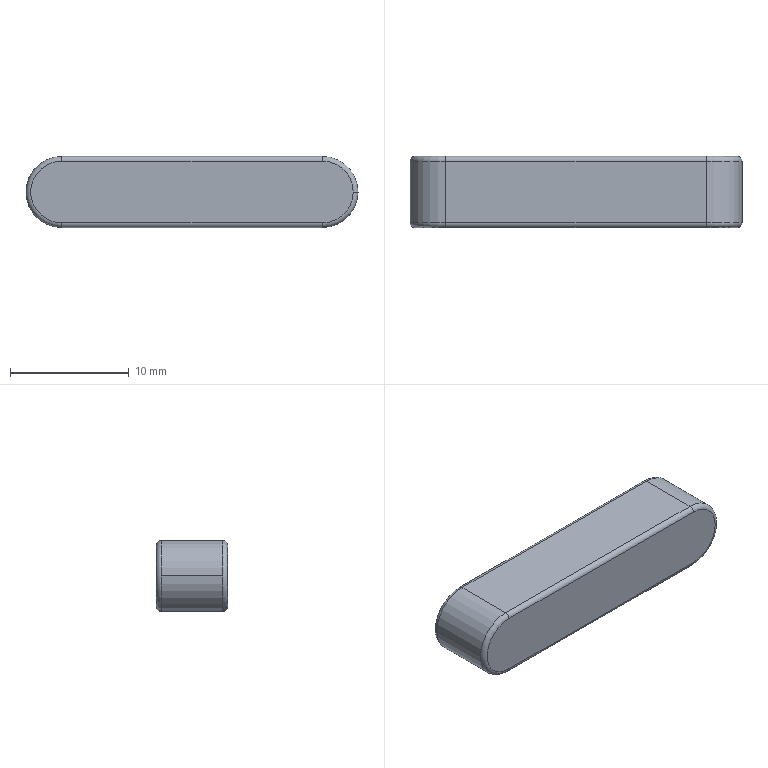Component | SolidWorks | XXXXX08-01-040514RotaryDriveShaft-1_6_28 A_T1096-1 | 1 solid | 17 faces | box 28 x 6 x 6 mm | volume 957 mm3 | cylinder 7 | torus 6 | plane 4 | commonest cylinder face diameters 0.8 x4 6 x3
build123d program:
from build123d import *

# Parameters (mm, degrees)
MATRIX_EXTRUDE_DEPTH = 6
FILLET1_R            = 0.4


with BuildPart() as part:
    # Sketch1 → Matrix-Extrude (new body)
    with BuildSketch(Plane.XY):
        with BuildLine():
            Line((-11, 3), (11, 3))
            ThreePointArc((11, 3), (14, 0), (11, -3))
            Line((11, -3), (-11, -3))
            ThreePointArc((-11, -3), (-14, 0), (-11, 3))
        make_face()
    extrude(amount=MATRIX_EXTRUDE_DEPTH)

    # Fillet1
    fillet1_edges = [part.edges().sort_by_distance(p)[0] for p in [
        (14, 0, 6),
        (0, 3, 6),
        (-14, 0, 6),
        (0, 3, 0),
        (14, 0, 0),
        (0, -3, 0),
        (-14, 0, 0),
        (0, -3, 6),
    ]]
    fillet(fillet1_edges, radius=FILLET1_R)


solid = part.part

# Placed as in the assembly
solid = solid.moved(Location((59.3, 13.5, 0), (90, 0, 0)))
STEP:
#1=CARTESIAN_POINT('',(2.87,0.5315,-0.));
#2=VERTEX_POINT('',#1);
#3=CARTESIAN_POINT('',(2.768,0.5315,-0.1024));
#4=VERTEX_POINT('',#3);
#5=CARTESIAN_POINT('',(2.768,0.5315,-0.));
#6=DIRECTION('',(0.,1.,0.));
#7=DIRECTION('',(1.,0.,-0.));
#8=AXIS2_PLACEMENT_3D('',#5,#6,#7);
#9=CIRCLE('',#8,0.1024);
#10=EDGE_CURVE('',#2,#4,#9,.T.);
#11=ORIENTED_EDGE('',*,*,#10,.F.);
#12=CARTESIAN_POINT('',(2.886,0.5157,-0.));
#13=VERTEX_POINT('',#12);
#14=CARTESIAN_POINT('',(2.87,0.5157,-0.));
#15=DIRECTION('',(-0.,0.,-1.));
#16=DIRECTION('',(-1.,0.,0.));
#17=AXIS2_PLACEMENT_3D('',#14,#15,#16);
#18=CIRCLE('',#17,0.01575);
#19=EDGE_CURVE('',#2,#13,#18,.T.);
#20=ORIENTED_EDGE('',*,*,#19,.T.);
#21=CARTESIAN_POINT('',(2.768,0.5157,-0.1181));
#22=VERTEX_POINT('',#21);
#23=CARTESIAN_POINT('',(2.768,0.5157,-0.));
#24=DIRECTION('',(0.,-1.,0.));
#25=DIRECTION('',(1.,0.,-0.));
#26=AXIS2_PLACEMENT_3D('',#23,#24,#25);
#27=CIRCLE('',#26,0.1181);
#28=EDGE_CURVE('',#22,#13,#27,.T.);
#29=ORIENTED_EDGE('',*,*,#28,.F.);
#30=CARTESIAN_POINT('',(2.768,0.5157,-0.1024));
#31=DIRECTION('',(1.,0.,-0.));
#32=DIRECTION('',(0.,1.,0.));
#33=AXIS2_PLACEMENT_3D('',#30,#31,#32);
#34=CIRCLE('',#33,0.01575);
#35=EDGE_CURVE('',#22,#4,#34,.T.);
#36=ORIENTED_EDGE('',*,*,#35,.T.);
#37=EDGE_LOOP('',(#11,#20,#29,#36));
#38=FACE_OUTER_BOUND('',#37,.T.);
#39=CARTESIAN_POINT('',(2.768,0.5157,-0.));
#40=DIRECTION('',(0.,-1.,0.));
#41=DIRECTION('',(1.,0.,-0.));
#42=AXIS2_PLACEMENT_3D('',#39,#40,#41);
#43=TOROIDAL_SURFACE('',#42,0.1024,0.01575);
#44=ADVANCED_FACE('',(#38),#43,.T.);
#45=CARTESIAN_POINT('',(2.886,0.311,-0.));
#46=VERTEX_POINT('',#45);
#47=CARTESIAN_POINT('',(2.768,0.311,-0.1181));
#48=VERTEX_POINT('',#47);
#49=CARTESIAN_POINT('',(2.768,0.311,-0.));
#50=DIRECTION('',(0.,1.,0.));
#51=DIRECTION('',(1.,0.,-0.));
#52=AXIS2_PLACEMENT_3D('',#49,#50,#51);
#53=CIRCLE('',#52,0.1181);
#54=EDGE_CURVE('',#46,#48,#53,.T.);
#55=ORIENTED_EDGE('',*,*,#54,.F.);
#56=CARTESIAN_POINT('',(2.87,0.2953,-0.));
#57=VERTEX_POINT('',#56);
#58=CARTESIAN_POINT('',(2.87,0.311,-0.));
#59=DIRECTION('',(-0.,0.,-1.));
#60=DIRECTION('',(-1.,0.,0.));
#61=AXIS2_PLACEMENT_3D('',#58,#59,#60);
#62=CIRCLE('',#61,0.01575);
#63=EDGE_CURVE('',#46,#57,#62,.T.);
#64=ORIENTED_EDGE('',*,*,#63,.T.);
#65=CARTESIAN_POINT('',(2.768,0.2953,-0.1024));
#66=VERTEX_POINT('',#65);
#67=CARTESIAN_POINT('',(2.768,0.2953,-0.));
#68=DIRECTION('',(0.,-1.,0.));
#69=DIRECTION('',(1.,0.,-0.));
#70=AXIS2_PLACEMENT_3D('',#67,#68,#69);
#71=CIRCLE('',#70,0.1024);
#72=EDGE_CURVE('',#66,#57,#71,.T.);
#73=ORIENTED_EDGE('',*,*,#72,.F.);
#74=CARTESIAN_POINT('',(2.768,0.311,-0.1024));
#75=DIRECTION('',(1.,0.,-0.));
#76=DIRECTION('',(0.,1.,0.));
#77=AXIS2_PLACEMENT_3D('',#74,#75,#76);
#78=CIRCLE('',#77,0.01575);
#79=EDGE_CURVE('',#66,#48,#78,.T.);
#80=ORIENTED_EDGE('',*,*,#79,.T.);
#81=EDGE_LOOP('',(#55,#64,#73,#80));
#82=FACE_OUTER_BOUND('',#81,.T.);
#83=CARTESIAN_POINT('',(2.768,0.311,-0.));
#84=DIRECTION('',(0.,-1.,0.));
#85=DIRECTION('',(1.,0.,-0.));
#86=AXIS2_PLACEMENT_3D('',#83,#84,#85);
#87=TOROIDAL_SURFACE('',#86,0.1024,0.01575);
#88=ADVANCED_FACE('',(#82),#87,.T.);
#89=CARTESIAN_POINT('',(1.902,0.311,-0.1181));
#90=VERTEX_POINT('',#89);
#91=CARTESIAN_POINT('',(1.783,0.311,-0.));
#92=VERTEX_POINT('',#91);
#93=CARTESIAN_POINT('',(1.902,0.311,-0.));
#94=DIRECTION('',(0.,1.,0.));
#95=DIRECTION('',(1.,0.,-0.));
#96=AXIS2_PLACEMENT_3D('',#93,#94,#95);
#97=CIRCLE('',#96,0.1181);
#98=EDGE_CURVE('',#90,#92,#97,.T.);
#99=ORIENTED_EDGE('',*,*,#98,.T.);
#100=CARTESIAN_POINT('',(1.783,0.5157,-0.));
#101=VERTEX_POINT('',#100);
#102=CARTESIAN_POINT('',(1.783,0.2953,-0.));
#103=DIRECTION('',(0.,1.,0.));
#104=VECTOR('',#103,39.37);
#105=LINE('',#102,#104);
#106=EDGE_CURVE('',#92,#101,#105,.T.);
#107=ORIENTED_EDGE('',*,*,#106,.T.);
#108=CARTESIAN_POINT('',(1.902,0.5157,-0.1181));
#109=VERTEX_POINT('',#108);
#110=CARTESIAN_POINT('',(1.902,0.5157,-0.));
#111=DIRECTION('',(0.,-1.,0.));
#112=DIRECTION('',(1.,0.,-0.));
#113=AXIS2_PLACEMENT_3D('',#110,#111,#112);
#114=CIRCLE('',#113,0.1181);
#115=EDGE_CURVE('',#101,#109,#114,.T.);
#116=ORIENTED_EDGE('',*,*,#115,.T.);
#117=CARTESIAN_POINT('',(1.902,0.2953,-0.1181));
#118=DIRECTION('',(0.,1.,0.));
#119=VECTOR('',#118,39.37);
#120=LINE('',#117,#119);
#121=EDGE_CURVE('',#90,#109,#120,.T.);
#122=ORIENTED_EDGE('',*,*,#121,.F.);
#123=EDGE_LOOP('',(#99,#107,#116,#122));
#124=FACE_OUTER_BOUND('',#123,.T.);
#125=CARTESIAN_POINT('',(1.902,0.2953,-0.));
#126=DIRECTION('',(0.,1.,0.));
#127=DIRECTION('',(-1.,0.,0.));
#128=AXIS2_PLACEMENT_3D('',#125,#126,#127);
#129=CYLINDRICAL_SURFACE('',#128,0.1181);
#130=ADVANCED_FACE('',(#124),#129,.T.);
#131=ORIENTED_EDGE('',*,*,#106,.F.);
#132=CARTESIAN_POINT('',(1.902,0.311,0.1181));
#133=VERTEX_POINT('',#132);
#134=CARTESIAN_POINT('',(1.902,0.311,-0.));
#135=DIRECTION('',(0.,1.,0.));
#136=DIRECTION('',(1.,0.,-0.));
#137=AXIS2_PLACEMENT_3D('',#134,#135,#136);
#138=CIRCLE('',#137,0.1181);
#139=EDGE_CURVE('',#92,#133,#138,.T.);
#140=ORIENTED_EDGE('',*,*,#139,.T.);
#141=CARTESIAN_POINT('',(1.902,0.5157,0.1181));
#142=VERTEX_POINT('',#141);
#143=CARTESIAN_POINT('',(1.902,0.2953,0.1181));
#144=DIRECTION('',(0.,1.,0.));
#145=VECTOR('',#144,39.37);
#146=LINE('',#143,#145);
#147=EDGE_CURVE('',#133,#142,#146,.T.);
#148=ORIENTED_EDGE('',*,*,#147,.T.);
#149=CARTESIAN_POINT('',(1.902,0.5157,-0.));
#150=DIRECTION('',(0.,-1.,0.));
#151=DIRECTION('',(1.,0.,-0.));
#152=AXIS2_PLACEMENT_3D('',#149,#150,#151);
#153=CIRCLE('',#152,0.1181);
#154=EDGE_CURVE('',#142,#101,#153,.T.);
#155=ORIENTED_EDGE('',*,*,#154,.T.);
#156=EDGE_LOOP('',(#131,#140,#148,#155));
#157=FACE_OUTER_BOUND('',#156,.T.);
#158=CARTESIAN_POINT('',(1.902,0.2953,-0.));
#159=DIRECTION('',(0.,1.,0.));
#160=DIRECTION('',(-1.,0.,0.));
#161=AXIS2_PLACEMENT_3D('',#158,#159,#160);
#162=CYLINDRICAL_SURFACE('',#161,0.1181);
#163=ADVANCED_FACE('',(#157),#162,.T.);
#164=CARTESIAN_POINT('',(2.768,0.2953,-0.1181));
#165=DIRECTION('',(0.,1.,0.));
#166=VECTOR('',#165,39.37);
#167=LINE('',#164,#166);
#168=EDGE_CURVE('',#48,#22,#167,.T.);
#169=ORIENTED_EDGE('',*,*,#168,.F.);
#170=CARTESIAN_POINT('',(1.902,0.311,-0.1181));
#171=DIRECTION('',(-1.,0.,0.));
#172=VECTOR('',#171,39.37);
#173=LINE('',#170,#172);
#174=EDGE_CURVE('',#48,#90,#173,.T.);
#175=ORIENTED_EDGE('',*,*,#174,.T.);
#176=ORIENTED_EDGE('',*,*,#121,.T.);
#177=CARTESIAN_POINT('',(1.902,0.5157,-0.1181));
#178=DIRECTION('',(1.,0.,-0.));
#179=VECTOR('',#178,39.37);
#180=LINE('',#177,#179);
#181=EDGE_CURVE('',#109,#22,#180,.T.);
#182=ORIENTED_EDGE('',*,*,#181,.T.);
#183=EDGE_LOOP('',(#169,#175,#176,#182));
#184=FACE_OUTER_BOUND('',#183,.T.);
#185=CARTESIAN_POINT('',(1.902,0.2953,-0.1181));
#186=DIRECTION('',(0.,0.,1.));
#187=DIRECTION('',(-1.,0.,0.));
#188=AXIS2_PLACEMENT_3D('',#185,#186,#187);
#189=PLANE('',#188);
#190=ADVANCED_FACE('',(#184),#189,.F.);
#191=CARTESIAN_POINT('',(2.768,0.311,0.1181));
#192=VERTEX_POINT('',#191);
#193=CARTESIAN_POINT('',(2.768,0.5157,0.1181));
#194=VERTEX_POINT('',#193);
#195=CARTESIAN_POINT('',(2.768,0.2953,0.1181));
#196=DIRECTION('',(0.,1.,0.));
#197=VECTOR('',#196,39.37);
#198=LINE('',#195,#197);
#199=EDGE_CURVE('',#192,#194,#198,.T.);
#200=ORIENTED_EDGE('',*,*,#199,.F.);
#201=CARTESIAN_POINT('',(2.768,0.311,-0.));
#202=DIRECTION('',(0.,1.,0.));
#203=DIRECTION('',(1.,0.,-0.));
#204=AXIS2_PLACEMENT_3D('',#201,#202,#203);
#205=CIRCLE('',#204,0.1181);
#206=EDGE_CURVE('',#192,#46,#205,.T.);
#207=ORIENTED_EDGE('',*,*,#206,.T.);
#208=ORIENTED_EDGE('',*,*,#54,.T.);
#209=ORIENTED_EDGE('',*,*,#168,.T.);
#210=ORIENTED_EDGE('',*,*,#28,.T.);
#211=CARTESIAN_POINT('',(2.768,0.5157,-0.));
#212=DIRECTION('',(0.,-1.,0.));
#213=DIRECTION('',(1.,0.,-0.));
#214=AXIS2_PLACEMENT_3D('',#211,#212,#213);
#215=CIRCLE('',#214,0.1181);
#216=EDGE_CURVE('',#13,#194,#215,.T.);
#217=ORIENTED_EDGE('',*,*,#216,.T.);
#218=EDGE_LOOP('',(#200,#207,#208,#209,#210,#217));
#219=FACE_OUTER_BOUND('',#218,.T.);
#220=CARTESIAN_POINT('',(2.768,0.2953,-0.));
#221=DIRECTION('',(0.,1.,0.));
#222=DIRECTION('',(-1.,0.,0.));
#223=AXIS2_PLACEMENT_3D('',#220,#221,#222);
#224=CYLINDRICAL_SURFACE('',#223,0.1181);
#225=ADVANCED_FACE('',(#219),#224,.T.);
#226=ORIENTED_EDGE('',*,*,#147,.F.);
#227=CARTESIAN_POINT('',(2.768,0.311,0.1181));
#228=DIRECTION('',(1.,0.,-0.));
#229=VECTOR('',#228,39.37);
#230=LINE('',#227,#229);
#231=EDGE_CURVE('',#133,#192,#230,.T.);
#232=ORIENTED_EDGE('',*,*,#231,.T.);
#233=ORIENTED_EDGE('',*,*,#199,.T.);
#234=CARTESIAN_POINT('',(1.902,0.5157,0.1181));
#235=DIRECTION('',(-1.,0.,0.));
#236=VECTOR('',#235,39.37);
#237=LINE('',#234,#236);
#238=EDGE_CURVE('',#194,#142,#237,.T.);
#239=ORIENTED_EDGE('',*,*,#238,.T.);
#240=EDGE_LOOP('',(#226,#232,#233,#239));
#241=FACE_OUTER_BOUND('',#240,.T.);
#242=CARTESIAN_POINT('',(1.902,0.2953,0.1181));
#243=DIRECTION('',(-0.,0.,-1.));
#244=DIRECTION('',(1.,0.,-0.));
#245=AXIS2_PLACEMENT_3D('',#242,#243,#244);
#246=PLANE('',#245);
#247=ADVANCED_FACE('',(#241),#246,.F.);
#248=CARTESIAN_POINT('',(1.902,0.2953,-0.1024));
#249=VERTEX_POINT('',#248);
#250=CARTESIAN_POINT('',(2.768,0.2953,-0.1024));
#251=DIRECTION('',(1.,0.,-0.));
#252=VECTOR('',#251,39.37);
#253=LINE('',#250,#252);
#254=EDGE_CURVE('',#249,#66,#253,.T.);
#255=ORIENTED_EDGE('',*,*,#254,.T.);
#256=ORIENTED_EDGE('',*,*,#72,.T.);
#257=CARTESIAN_POINT('',(2.768,0.2953,0.1024));
#258=VERTEX_POINT('',#257);
#259=CARTESIAN_POINT('',(2.768,0.2953,-0.));
#260=DIRECTION('',(0.,-1.,0.));
#261=DIRECTION('',(1.,0.,-0.));
#262=AXIS2_PLACEMENT_3D('',#259,#260,#261);
#263=CIRCLE('',#262,0.1024);
#264=EDGE_CURVE('',#57,#258,#263,.T.);
#265=ORIENTED_EDGE('',*,*,#264,.T.);
#266=CARTESIAN_POINT('',(1.902,0.2953,0.1024));
#267=VERTEX_POINT('',#266);
#268=CARTESIAN_POINT('',(1.902,0.2953,0.1024));
#269=DIRECTION('',(-1.,0.,0.));
#270=VECTOR('',#269,39.37);
#271=LINE('',#268,#270);
#272=EDGE_CURVE('',#258,#267,#271,.T.);
#273=ORIENTED_EDGE('',*,*,#272,.T.);
#274=CARTESIAN_POINT('',(1.902,0.2953,-0.));
#275=DIRECTION('',(0.,-1.,0.));
#276=DIRECTION('',(1.,0.,-0.));
#277=AXIS2_PLACEMENT_3D('',#274,#275,#276);
#278=CIRCLE('',#277,0.1024);
#279=EDGE_CURVE('',#267,#249,#278,.T.);
#280=ORIENTED_EDGE('',*,*,#279,.T.);
#281=EDGE_LOOP('',(#255,#256,#265,#273,#280));
#282=FACE_OUTER_BOUND('',#281,.T.);
#283=CARTESIAN_POINT('',(1.902,0.2953,-0.));
#284=DIRECTION('',(0.,-1.,0.));
#285=DIRECTION('',(1.,0.,-0.));
#286=AXIS2_PLACEMENT_3D('',#283,#284,#285);
#287=PLANE('',#286);
#288=ADVANCED_FACE('',(#282),#287,.T.);
#289=CARTESIAN_POINT('',(1.902,0.5315,0.1024));
#290=VERTEX_POINT('',#289);
#291=CARTESIAN_POINT('',(2.768,0.5315,0.1024));
#292=VERTEX_POINT('',#291);
#293=CARTESIAN_POINT('',(1.902,0.5315,0.1024));
#294=DIRECTION('',(1.,0.,-0.));
#295=VECTOR('',#294,39.37);
#296=LINE('',#293,#295);
#297=EDGE_CURVE('',#290,#292,#296,.T.);
#298=ORIENTED_EDGE('',*,*,#297,.T.);
#299=CARTESIAN_POINT('',(2.768,0.5315,-0.));
#300=DIRECTION('',(0.,1.,0.));
#301=DIRECTION('',(1.,0.,-0.));
#302=AXIS2_PLACEMENT_3D('',#299,#300,#301);
#303=CIRCLE('',#302,0.1024);
#304=EDGE_CURVE('',#292,#2,#303,.T.);
#305=ORIENTED_EDGE('',*,*,#304,.T.);
#306=ORIENTED_EDGE('',*,*,#10,.T.);
#307=CARTESIAN_POINT('',(1.902,0.5315,-0.1024));
#308=VERTEX_POINT('',#307);
#309=CARTESIAN_POINT('',(1.902,0.5315,-0.1024));
#310=DIRECTION('',(-1.,0.,0.));
#311=VECTOR('',#310,39.37);
#312=LINE('',#309,#311);
#313=EDGE_CURVE('',#4,#308,#312,.T.);
#314=ORIENTED_EDGE('',*,*,#313,.T.);
#315=CARTESIAN_POINT('',(1.902,0.5315,-0.));
#316=DIRECTION('',(0.,1.,0.));
#317=DIRECTION('',(1.,0.,-0.));
#318=AXIS2_PLACEMENT_3D('',#315,#316,#317);
#319=CIRCLE('',#318,0.1024);
#320=EDGE_CURVE('',#308,#290,#319,.T.);
#321=ORIENTED_EDGE('',*,*,#320,.T.);
#322=EDGE_LOOP('',(#298,#305,#306,#314,#321));
#323=FACE_OUTER_BOUND('',#322,.T.);
#324=CARTESIAN_POINT('',(1.902,0.5315,-0.));
#325=DIRECTION('',(0.,-1.,0.));
#326=DIRECTION('',(1.,0.,-0.));
#327=AXIS2_PLACEMENT_3D('',#324,#325,#326);
#328=PLANE('',#327);
#329=ADVANCED_FACE('',(#323),#328,.F.);
#330=CARTESIAN_POINT('',(1.902,0.311,0.1024));
#331=DIRECTION('',(1.,0.,-0.));
#332=DIRECTION('',(0.,1.,0.));
#333=AXIS2_PLACEMENT_3D('',#330,#331,#332);
#334=CIRCLE('',#333,0.01575);
#335=EDGE_CURVE('',#133,#267,#334,.T.);
#336=ORIENTED_EDGE('',*,*,#335,.F.);
#337=ORIENTED_EDGE('',*,*,#139,.F.);
#338=ORIENTED_EDGE('',*,*,#98,.F.);
#339=CARTESIAN_POINT('',(1.902,0.311,-0.1024));
#340=DIRECTION('',(1.,0.,-0.));
#341=DIRECTION('',(0.,1.,0.));
#342=AXIS2_PLACEMENT_3D('',#339,#340,#341);
#343=CIRCLE('',#342,0.01575);
#344=EDGE_CURVE('',#249,#90,#343,.T.);
#345=ORIENTED_EDGE('',*,*,#344,.F.);
#346=ORIENTED_EDGE('',*,*,#279,.F.);
#347=EDGE_LOOP('',(#336,#337,#338,#345,#346));
#348=FACE_OUTER_BOUND('',#347,.T.);
#349=CARTESIAN_POINT('',(1.902,0.311,-0.));
#350=DIRECTION('',(0.,-1.,0.));
#351=DIRECTION('',(1.,0.,-0.));
#352=AXIS2_PLACEMENT_3D('',#349,#350,#351);
#353=TOROIDAL_SURFACE('',#352,0.1024,0.01575);
#354=ADVANCED_FACE('',(#348),#353,.T.);
#355=ORIENTED_EDGE('',*,*,#344,.T.);
#356=ORIENTED_EDGE('',*,*,#174,.F.);
#357=ORIENTED_EDGE('',*,*,#79,.F.);
#358=ORIENTED_EDGE('',*,*,#254,.F.);
#359=EDGE_LOOP('',(#355,#356,#357,#358));
#360=FACE_OUTER_BOUND('',#359,.T.);
#361=CARTESIAN_POINT('',(1.902,0.311,-0.1024));
#362=DIRECTION('',(-1.,0.,0.));
#363=DIRECTION('',(0.,0.,-1.));
#364=AXIS2_PLACEMENT_3D('',#361,#362,#363);
#365=CYLINDRICAL_SURFACE('',#364,0.01575);
#366=ADVANCED_FACE('',(#360),#365,.T.);
#367=ORIENTED_EDGE('',*,*,#335,.T.);
#368=ORIENTED_EDGE('',*,*,#272,.F.);
#369=CARTESIAN_POINT('',(2.768,0.311,0.1024));
#370=DIRECTION('',(1.,0.,-0.));
#371=DIRECTION('',(0.,1.,0.));
#372=AXIS2_PLACEMENT_3D('',#369,#370,#371);
#373=CIRCLE('',#372,0.01575);
#374=EDGE_CURVE('',#192,#258,#373,.T.);
#375=ORIENTED_EDGE('',*,*,#374,.F.);
#376=ORIENTED_EDGE('',*,*,#231,.F.);
#377=EDGE_LOOP('',(#367,#368,#375,#376));
#378=FACE_OUTER_BOUND('',#377,.T.);
#379=CARTESIAN_POINT('',(1.902,0.311,0.1024));
#380=DIRECTION('',(1.,0.,-0.));
#381=DIRECTION('',(0.,0.,1.));
#382=AXIS2_PLACEMENT_3D('',#379,#380,#381);
#383=CYLINDRICAL_SURFACE('',#382,0.01575);
#384=ADVANCED_FACE('',(#378),#383,.T.);
#385=ORIENTED_EDGE('',*,*,#63,.F.);
#386=ORIENTED_EDGE('',*,*,#206,.F.);
#387=ORIENTED_EDGE('',*,*,#374,.T.);
#388=ORIENTED_EDGE('',*,*,#264,.F.);
#389=EDGE_LOOP('',(#385,#386,#387,#388));
#390=FACE_OUTER_BOUND('',#389,.T.);
#391=CARTESIAN_POINT('',(2.768,0.311,-0.));
#392=DIRECTION('',(0.,-1.,0.));
#393=DIRECTION('',(1.,0.,-0.));
#394=AXIS2_PLACEMENT_3D('',#391,#392,#393);
#395=TOROIDAL_SURFACE('',#394,0.1024,0.01575);
#396=ADVANCED_FACE('',(#390),#395,.T.);
#397=CARTESIAN_POINT('',(1.902,0.5157,0.1024));
#398=DIRECTION('',(1.,0.,-0.));
#399=DIRECTION('',(0.,1.,0.));
#400=AXIS2_PLACEMENT_3D('',#397,#398,#399);
#401=CIRCLE('',#400,0.01575);
#402=EDGE_CURVE('',#290,#142,#401,.T.);
#403=ORIENTED_EDGE('',*,*,#402,.F.);
#404=ORIENTED_EDGE('',*,*,#320,.F.);
#405=CARTESIAN_POINT('',(1.902,0.5157,-0.1024));
#406=DIRECTION('',(1.,0.,-0.));
#407=DIRECTION('',(0.,1.,0.));
#408=AXIS2_PLACEMENT_3D('',#405,#406,#407);
#409=CIRCLE('',#408,0.01575);
#410=EDGE_CURVE('',#109,#308,#409,.T.);
#411=ORIENTED_EDGE('',*,*,#410,.F.);
#412=ORIENTED_EDGE('',*,*,#115,.F.);
#413=ORIENTED_EDGE('',*,*,#154,.F.);
#414=EDGE_LOOP('',(#403,#404,#411,#412,#413));
#415=FACE_OUTER_BOUND('',#414,.T.);
#416=CARTESIAN_POINT('',(1.902,0.5157,-0.));
#417=DIRECTION('',(0.,-1.,0.));
#418=DIRECTION('',(1.,0.,-0.));
#419=AXIS2_PLACEMENT_3D('',#416,#417,#418);
#420=TOROIDAL_SURFACE('',#419,0.1024,0.01575);
#421=ADVANCED_FACE('',(#415),#420,.T.);
#422=ORIENTED_EDGE('',*,*,#410,.T.);
#423=ORIENTED_EDGE('',*,*,#313,.F.);
#424=ORIENTED_EDGE('',*,*,#35,.F.);
#425=ORIENTED_EDGE('',*,*,#181,.F.);
#426=EDGE_LOOP('',(#422,#423,#424,#425));
#427=FACE_OUTER_BOUND('',#426,.T.);
#428=CARTESIAN_POINT('',(1.902,0.5157,-0.1024));
#429=DIRECTION('',(1.,0.,-0.));
#430=DIRECTION('',(0.,0.,1.));
#431=AXIS2_PLACEMENT_3D('',#428,#429,#430);
#432=CYLINDRICAL_SURFACE('',#431,0.01575);
#433=ADVANCED_FACE('',(#427),#432,.T.);
#434=ORIENTED_EDGE('',*,*,#402,.T.);
#435=ORIENTED_EDGE('',*,*,#238,.F.);
#436=CARTESIAN_POINT('',(2.768,0.5157,0.1024));
#437=DIRECTION('',(1.,0.,-0.));
#438=DIRECTION('',(0.,1.,0.));
#439=AXIS2_PLACEMENT_3D('',#436,#437,#438);
#440=CIRCLE('',#439,0.01575);
#441=EDGE_CURVE('',#292,#194,#440,.T.);
#442=ORIENTED_EDGE('',*,*,#441,.F.);
#443=ORIENTED_EDGE('',*,*,#297,.F.);
#444=EDGE_LOOP('',(#434,#435,#442,#443));
#445=FACE_OUTER_BOUND('',#444,.T.);
#446=CARTESIAN_POINT('',(1.902,0.5157,0.1024));
#447=DIRECTION('',(-1.,0.,0.));
#448=DIRECTION('',(0.,0.,-1.));
#449=AXIS2_PLACEMENT_3D('',#446,#447,#448);
#450=CYLINDRICAL_SURFACE('',#449,0.01575);
#451=ADVANCED_FACE('',(#445),#450,.T.);
#452=ORIENTED_EDGE('',*,*,#19,.F.);
#453=ORIENTED_EDGE('',*,*,#304,.F.);
#454=ORIENTED_EDGE('',*,*,#441,.T.);
#455=ORIENTED_EDGE('',*,*,#216,.F.);
#456=EDGE_LOOP('',(#452,#453,#454,#455));
#457=FACE_OUTER_BOUND('',#456,.T.);
#458=CARTESIAN_POINT('',(2.768,0.5157,-0.));
#459=DIRECTION('',(0.,-1.,0.));
#460=DIRECTION('',(1.,0.,-0.));
#461=AXIS2_PLACEMENT_3D('',#458,#459,#460);
#462=TOROIDAL_SURFACE('',#461,0.1024,0.01575);
#463=ADVANCED_FACE('',(#457),#462,.T.);
#464=CLOSED_SHELL('',(#44,#88,#130,#163,#190,#225,#247,#288,#329,#354,#366,#384,#396,#421,#433,#451,#463));
#465=MANIFOLD_SOLID_BREP('',#464);
#466=CARTESIAN_POINT('',(0.,0.,0.));
#467=DIRECTION('',(0.,0.,1.));
#468=DIRECTION('',(1.,0.,0.));
#469=AXIS2_PLACEMENT_3D('',#466,#467,#468);
#470=(LENGTH_UNIT()NAMED_UNIT(*)SI_UNIT($,.METRE.));
#471=LENGTH_MEASURE_WITH_UNIT(LENGTH_MEASURE(0.0254),#470);
#472=DIMENSIONAL_EXPONENTS(1.,0.,0.,0.,0.,0.,0.);
#473=(CONVERSION_BASED_UNIT('',#471)LENGTH_UNIT()NAMED_UNIT(#472));
#474=UNCERTAINTY_MEASURE_WITH_UNIT(LENGTH_MEASURE(0.00001),#473,'','');
#475=(NAMED_UNIT(*)PLANE_ANGLE_UNIT()SI_UNIT($,.RADIAN.));
#476=(NAMED_UNIT(*)SI_UNIT($,.STERADIAN.)SOLID_ANGLE_UNIT());
#477=(GEOMETRIC_REPRESENTATION_CONTEXT(3)GLOBAL_UNCERTAINTY_ASSIGNED_CONTEXT((#474))GLOBAL_UNIT_ASSIGNED_CONTEXT((#473,#475,#476))REPRESENTATION_CONTEXT('',''));
#478=ADVANCED_BREP_SHAPE_REPRESENTATION('',(#465,#469),#477);
#479=COLOUR_RGB('',0.7922,0.8196,0.9333);
#480=FILL_AREA_STYLE_COLOUR('',#479);
#481=FILL_AREA_STYLE('',(#480));
#482=SURFACE_STYLE_FILL_AREA(#481);
#483=SURFACE_SIDE_STYLE('',(#482));
#484=SURFACE_STYLE_USAGE(.BOTH.,#483);
#485=PRESENTATION_STYLE_ASSIGNMENT((#484));
#486=STYLED_ITEM('',(#485),#465);
#487=PRESENTATION_LAYER_ASSIGNMENT('','',(#486));
#488=(LENGTH_UNIT()NAMED_UNIT(*)SI_UNIT($,.METRE.));
#489=LENGTH_MEASURE_WITH_UNIT(LENGTH_MEASURE(0.0254),#488);
#490=DIMENSIONAL_EXPONENTS(1.,0.,0.,0.,0.,0.,0.);
#491=(CONVERSION_BASED_UNIT('',#489)LENGTH_UNIT()NAMED_UNIT(#490));
#492=UNCERTAINTY_MEASURE_WITH_UNIT(LENGTH_MEASURE(0.00001),#491,'','');
#493=(NAMED_UNIT(*)PLANE_ANGLE_UNIT()SI_UNIT($,.RADIAN.));
#494=(NAMED_UNIT(*)SI_UNIT($,.STERADIAN.)SOLID_ANGLE_UNIT());
#495=(GEOMETRIC_REPRESENTATION_CONTEXT(3)GLOBAL_UNCERTAINTY_ASSIGNED_CONTEXT((#492))GLOBAL_UNIT_ASSIGNED_CONTEXT((#491,#493,#494))REPRESENTATION_CONTEXT('',''));
#496=MECHANICAL_DESIGN_GEOMETRIC_PRESENTATION_REPRESENTATION('',(#486),#495);